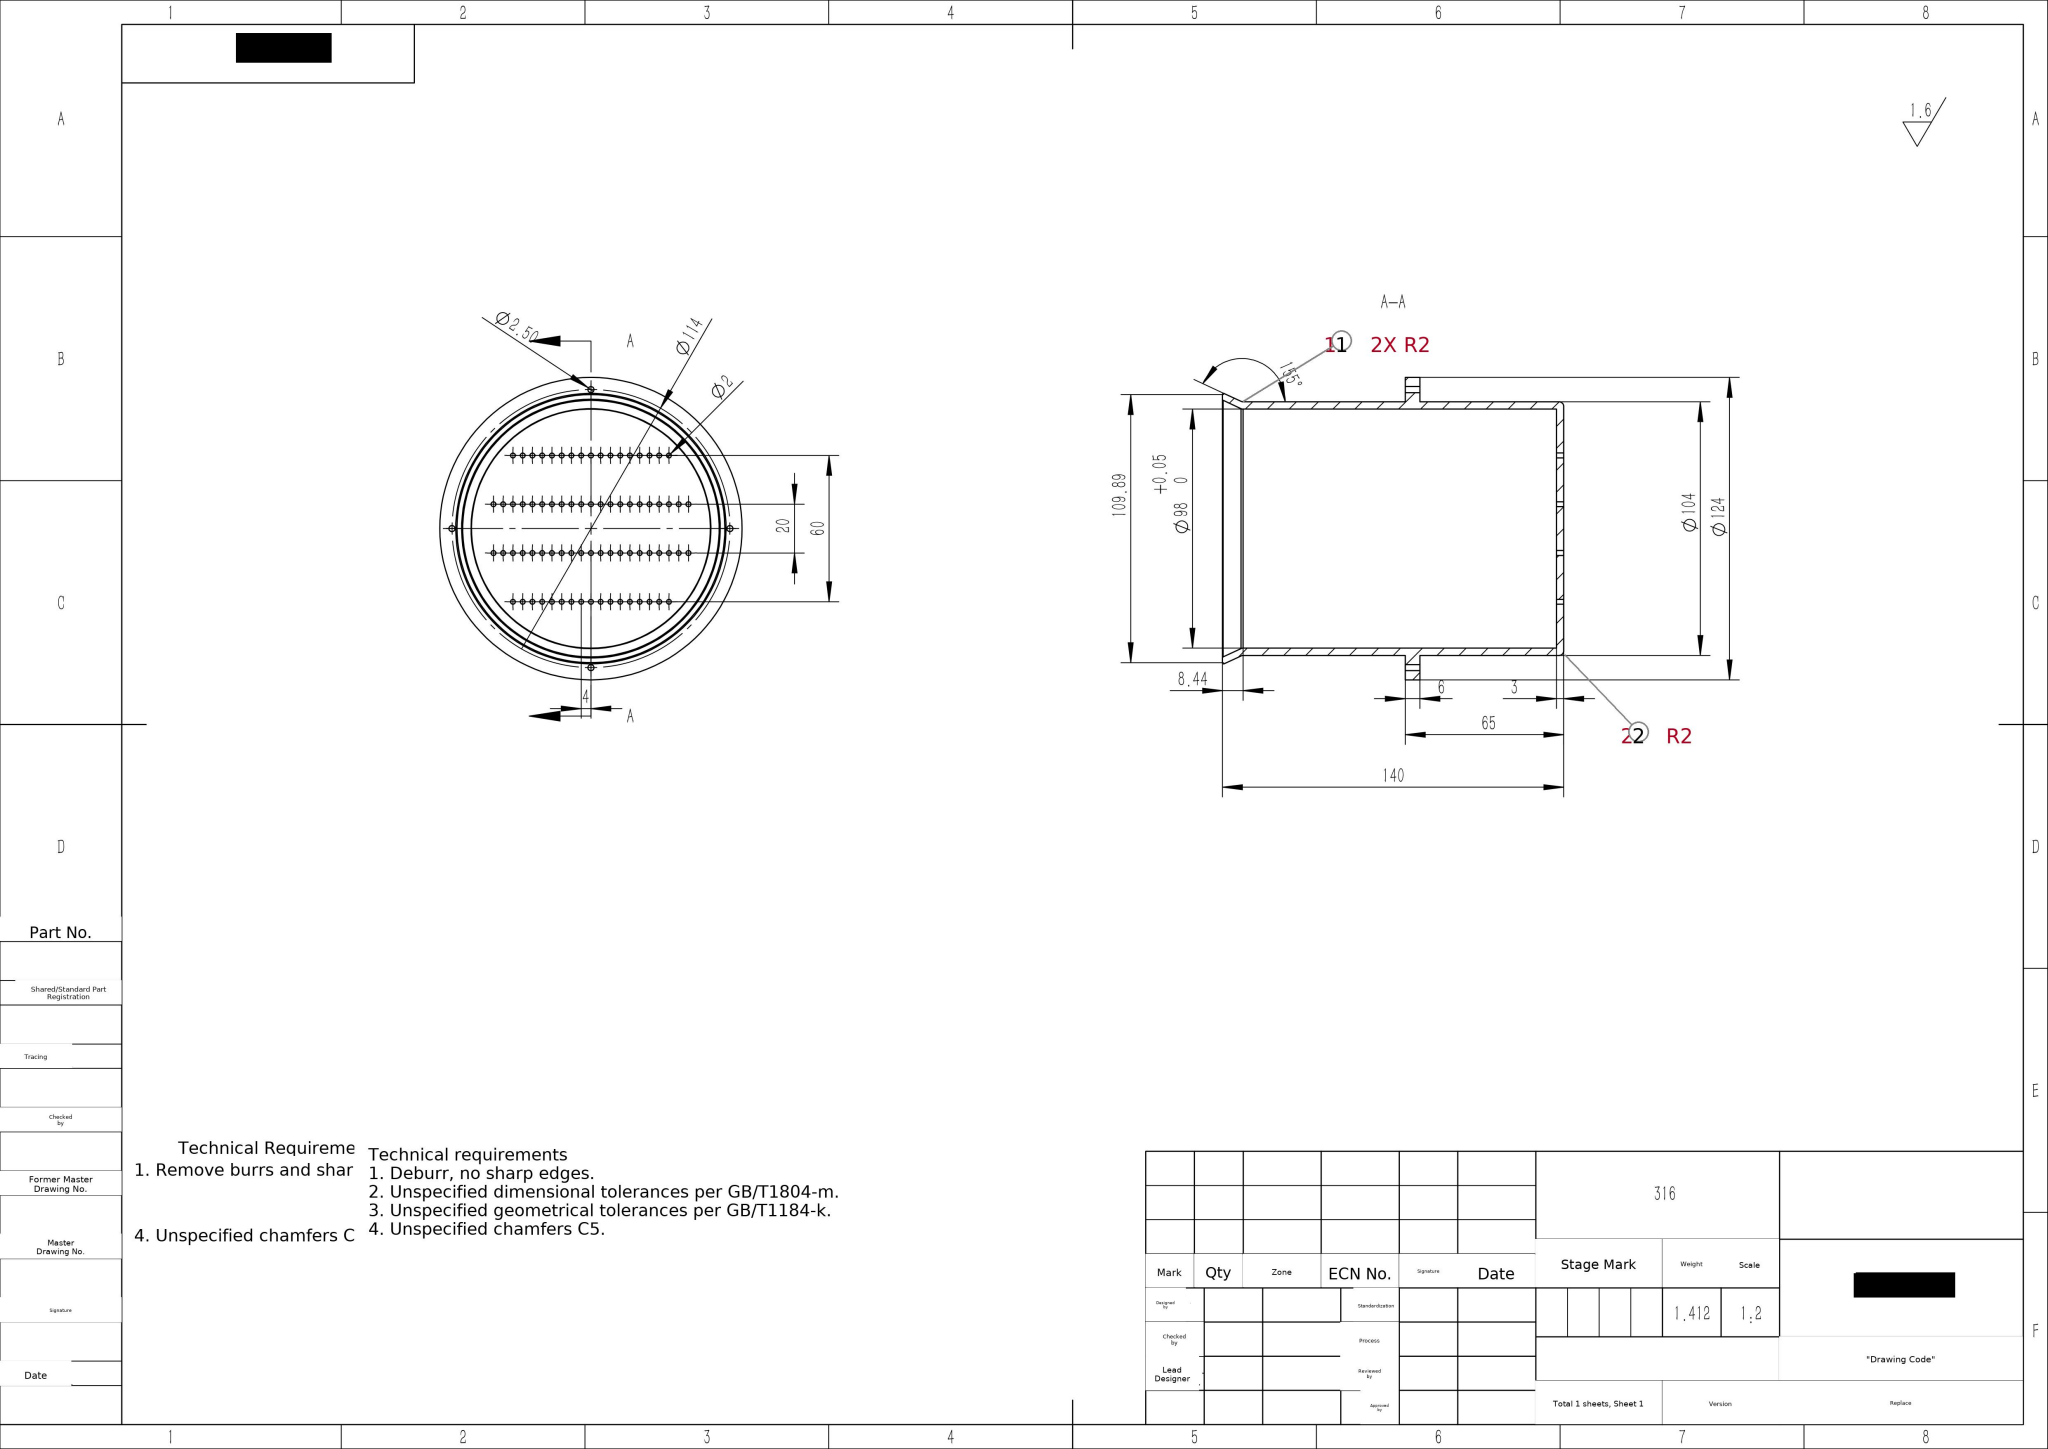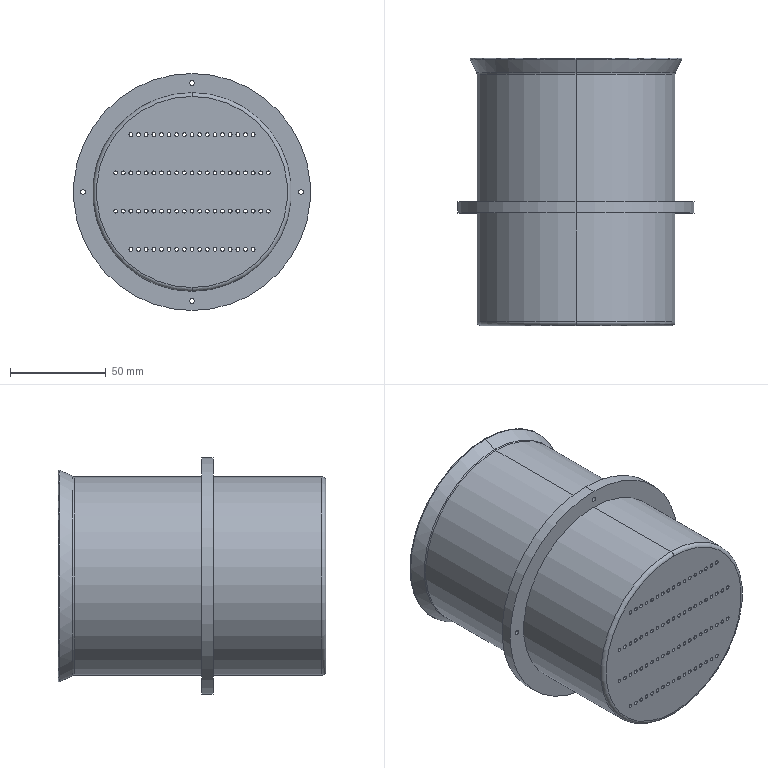Part | SolidWorks | mm | material 316 | 1 solid | 187 faces | box 124 x 140 x 124 mm | volume 176498 mm3 | cylinder 168 | torus 10 | plane 5 | cone 4 | commonest cylinder face diameters 2 x152 2.5 x8 104 x4 124 x2 98 x2